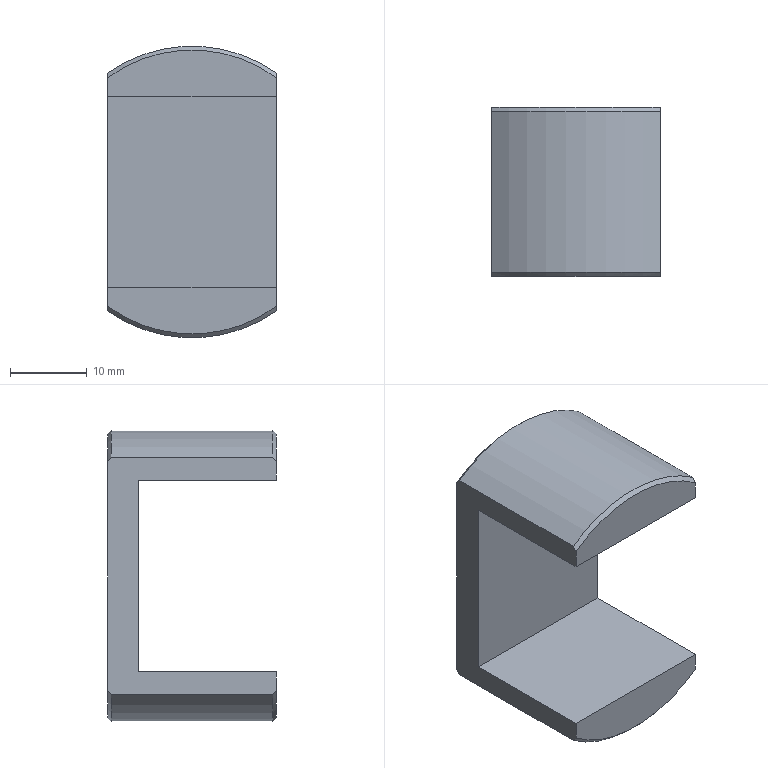Component | NX | LARGE_SLIDER | 1 solid | 14 faces | box 22 x 22 x 38 mm | volume 7394 mm3 | plane 8 | cone 4 | cylinder 2 | commonest cylinder face diameters 38 x2
STEP:
#1=CARTESIAN_POINT('',(0.,0.,0.));
#2=DIRECTION('',(0.,0.,1.));
#3=DIRECTION('',(1.,0.,0.));
#4=AXIS2_PLACEMENT_3D('',#1,#2,#3);
#5=CARTESIAN_POINT('',(-11.,-32.,-10.374));
#6=VERTEX_POINT('',#5);
#7=CARTESIAN_POINT('',(-11.,-32.,-8.));
#8=VERTEX_POINT('',#7);
#9=CARTESIAN_POINT('',(-11.,-32.,-10.992));
#10=DIRECTION('',(0.,0.,1.));
#11=VECTOR('',#10,1.);
#12=LINE('',#9,#11);
#13=CARTESIAN_POINT('',(0.,-32.,4.5));
#14=DIRECTION('',(0.,-1.,0.));
#15=DIRECTION('',(1.,0.,0.));
#16=AXIS2_PLACEMENT_3D('',#13,#14,#15);
#17=PLANE('',#16);
#18=CARTESIAN_POINT('',(-11.,-15.492));
#19=DIRECTION('',(0.,1.));
#20=VECTOR('',#19,1.);
#21=LINE('',#18,#20);
#22=(GEOMETRIC_REPRESENTATION_CONTEXT(2)PARAMETRIC_REPRESENTATION_CONTEXT()REPRESENTATION_CONTEXT('',''));
#23=DEFINITIONAL_REPRESENTATION('',(#21),#22);
#24=PCURVE('',#17,#23);
#25=CARTESIAN_POINT('',(-11.,-7.,-10.992));
#26=DIRECTION('',(1.,0.,0.));
#27=DIRECTION('',(0.,1.,0.));
#28=AXIS2_PLACEMENT_3D('',#25,#26,#27);
#29=PLANE('',#28);
#30=CARTESIAN_POINT('',(-25.,0.));
#31=DIRECTION('',(0.,1.));
#32=VECTOR('',#31,1.);
#33=LINE('',#30,#32);
#34=(GEOMETRIC_REPRESENTATION_CONTEXT(2)PARAMETRIC_REPRESENTATION_CONTEXT()REPRESENTATION_CONTEXT('',''));
#35=DEFINITIONAL_REPRESENTATION('',(#33),#34);
#36=PCURVE('',#29,#35);
#37=SURFACE_CURVE('',#12,(#24,#36),.PCURVE_S1.);
#38=EDGE_CURVE('',#6,#8,#37,.T.);
#39=ORIENTED_EDGE('',*,*,#38,.F.);
#40=CARTESIAN_POINT('',(11.,-32.,-10.374));
#41=VERTEX_POINT('',#40);
#42=CARTESIAN_POINT('',(0.,-32.,4.5));
#43=DIRECTION('',(0.,-1.,0.));
#44=DIRECTION('',(1.,0.,0.));
#45=AXIS2_PLACEMENT_3D('',#42,#43,#44);
#46=CIRCLE('',#45,18.5);
#47=CARTESIAN_POINT('',(0.,0.));
#48=DIRECTION('',(1.,0.));
#49=AXIS2_PLACEMENT_2D('',#47,#48);
#50=CIRCLE('',#49,18.5);
#51=(GEOMETRIC_REPRESENTATION_CONTEXT(2)PARAMETRIC_REPRESENTATION_CONTEXT()REPRESENTATION_CONTEXT('',''));
#52=DEFINITIONAL_REPRESENTATION('',(#50),#51);
#53=PCURVE('',#17,#52);
#54=CARTESIAN_POINT('',(0.,-31.5,4.5));
#55=DIRECTION('',(0.,1.,0.));
#56=DIRECTION('',(-1.,0.,0.));
#57=AXIS2_PLACEMENT_3D('',#54,#55,#56);
#58=CONICAL_SURFACE('',#57,19.,0.7854);
#59=CARTESIAN_POINT('',(9.425,-0.5));
#60=DIRECTION('',(-1.,0.));
#61=VECTOR('',#60,1.);
#62=LINE('',#59,#61);
#63=(GEOMETRIC_REPRESENTATION_CONTEXT(2)PARAMETRIC_REPRESENTATION_CONTEXT()REPRESENTATION_CONTEXT('',''));
#64=DEFINITIONAL_REPRESENTATION('',(#62),#63);
#65=PCURVE('',#58,#64);
#66=SURFACE_CURVE('',#46,(#53,#65),.PCURVE_S1.);
#67=EDGE_CURVE('',#6,#41,#66,.T.);
#68=ORIENTED_EDGE('',*,*,#67,.T.);
#69=CARTESIAN_POINT('',(11.,-32.,-8.));
#70=VERTEX_POINT('',#69);
#71=CARTESIAN_POINT('',(11.,-32.,19.992));
#72=DIRECTION('',(0.,0.,-1.));
#73=VECTOR('',#72,1.);
#74=LINE('',#71,#73);
#75=CARTESIAN_POINT('',(11.,15.492));
#76=DIRECTION('',(0.,-1.));
#77=VECTOR('',#76,1.);
#78=LINE('',#75,#77);
#79=(GEOMETRIC_REPRESENTATION_CONTEXT(2)PARAMETRIC_REPRESENTATION_CONTEXT()REPRESENTATION_CONTEXT('',''));
#80=DEFINITIONAL_REPRESENTATION('',(#78),#79);
#81=PCURVE('',#17,#80);
#82=CARTESIAN_POINT('',(11.,-7.,19.992));
#83=DIRECTION('',(-1.,0.,0.));
#84=DIRECTION('',(0.,-1.,0.));
#85=AXIS2_PLACEMENT_3D('',#82,#83,#84);
#86=PLANE('',#85);
#87=CARTESIAN_POINT('',(25.,0.));
#88=DIRECTION('',(0.,-1.));
#89=VECTOR('',#88,1.);
#90=LINE('',#87,#89);
#91=(GEOMETRIC_REPRESENTATION_CONTEXT(2)PARAMETRIC_REPRESENTATION_CONTEXT()REPRESENTATION_CONTEXT('',''));
#92=DEFINITIONAL_REPRESENTATION('',(#90),#91);
#93=PCURVE('',#86,#92);
#94=SURFACE_CURVE('',#74,(#81,#93),.PCURVE_S1.);
#95=EDGE_CURVE('',#70,#41,#94,.T.);
#96=ORIENTED_EDGE('',*,*,#95,.F.);
#97=CARTESIAN_POINT('',(21.,-32.,-8.));
#98=DIRECTION('',(-1.,0.,0.));
#99=VECTOR('',#98,1.);
#100=LINE('',#97,#99);
#101=CARTESIAN_POINT('',(21.,-12.5));
#102=DIRECTION('',(-1.,0.));
#103=VECTOR('',#102,1.);
#104=LINE('',#101,#103);
#105=(GEOMETRIC_REPRESENTATION_CONTEXT(2)PARAMETRIC_REPRESENTATION_CONTEXT()REPRESENTATION_CONTEXT('',''));
#106=DEFINITIONAL_REPRESENTATION('',(#104),#105);
#107=PCURVE('',#17,#106);
#108=CARTESIAN_POINT('',(21.,-14.,-8.));
#109=DIRECTION('',(0.,0.,-1.));
#110=DIRECTION('',(0.,1.,0.));
#111=AXIS2_PLACEMENT_3D('',#108,#109,#110);
#112=PLANE('',#111);
#113=CARTESIAN_POINT('',(-18.,0.));
#114=DIRECTION('',(0.,-1.));
#115=VECTOR('',#114,1.);
#116=LINE('',#113,#115);
#117=(GEOMETRIC_REPRESENTATION_CONTEXT(2)PARAMETRIC_REPRESENTATION_CONTEXT()REPRESENTATION_CONTEXT('',''));
#118=DEFINITIONAL_REPRESENTATION('',(#116),#117);
#119=PCURVE('',#112,#118);
#120=SURFACE_CURVE('',#100,(#107,#119),.PCURVE_S1.);
#121=EDGE_CURVE('',#70,#8,#120,.T.);
#122=ORIENTED_EDGE('',*,*,#121,.T.);
#123=EDGE_LOOP('',(#39,#68,#96,#122));
#124=FACE_BOUND('',#123,.T.);
#125=ADVANCED_FACE('',(#124),#17,.T.);
#126=CARTESIAN_POINT('',(-11.,-10.5,-10.992));
#127=VERTEX_POINT('',#126);
#128=CARTESIAN_POINT('',(-11.,-31.5,-10.992));
#129=VERTEX_POINT('',#128);
#130=CARTESIAN_POINT('',(-11.,-7.,-10.992));
#131=DIRECTION('',(0.,-1.,0.));
#132=VECTOR('',#131,1.);
#133=LINE('',#130,#132);
#134=CARTESIAN_POINT('',(0.,-10.,4.5));
#135=DIRECTION('',(0.,-1.,0.));
#136=DIRECTION('',(1.,0.,0.));
#137=AXIS2_PLACEMENT_3D('',#134,#135,#136);
#138=CYLINDRICAL_SURFACE('',#137,19.);
#139=CARTESIAN_POINT('',(4.095,-3.));
#140=DIRECTION('',(0.,1.));
#141=VECTOR('',#140,1.);
#142=LINE('',#139,#141);
#143=(GEOMETRIC_REPRESENTATION_CONTEXT(2)PARAMETRIC_REPRESENTATION_CONTEXT()REPRESENTATION_CONTEXT('',''));
#144=DEFINITIONAL_REPRESENTATION('',(#142),#143);
#145=PCURVE('',#138,#144);
#146=CARTESIAN_POINT('',(0.,0.));
#147=DIRECTION('',(-1.,0.));
#148=VECTOR('',#147,1.);
#149=LINE('',#146,#148);
#150=(GEOMETRIC_REPRESENTATION_CONTEXT(2)PARAMETRIC_REPRESENTATION_CONTEXT()REPRESENTATION_CONTEXT('',''));
#151=DEFINITIONAL_REPRESENTATION('',(#149),#150);
#152=PCURVE('',#29,#151);
#153=SURFACE_CURVE('',#133,(#145,#152),.PCURVE_S1.);
#154=EDGE_CURVE('',#127,#129,#153,.T.);
#155=ORIENTED_EDGE('',*,*,#154,.F.);
#156=CARTESIAN_POINT('',(11.,-10.5,-10.992));
#157=VERTEX_POINT('',#156);
#158=CARTESIAN_POINT('',(0.,-10.5,4.5));
#159=DIRECTION('',(0.,-1.,0.));
#160=DIRECTION('',(-1.,0.,0.));
#161=AXIS2_PLACEMENT_3D('',#158,#159,#160);
#162=CIRCLE('',#161,19.);
#163=CARTESIAN_POINT('',(3.142,0.5));
#164=DIRECTION('',(1.,0.));
#165=VECTOR('',#164,1.);
#166=LINE('',#163,#165);
#167=(GEOMETRIC_REPRESENTATION_CONTEXT(2)PARAMETRIC_REPRESENTATION_CONTEXT()REPRESENTATION_CONTEXT('',''));
#168=DEFINITIONAL_REPRESENTATION('',(#166),#167);
#169=PCURVE('',#138,#168);
#170=CARTESIAN_POINT('',(0.,-10.5,4.5));
#171=DIRECTION('',(0.,-1.,0.));
#172=DIRECTION('',(1.,0.,0.));
#173=AXIS2_PLACEMENT_3D('',#170,#171,#172);
#174=CONICAL_SURFACE('',#173,19.,0.7854);
#175=CARTESIAN_POINT('',(3.142,0.));
#176=DIRECTION('',(1.,-0.));
#177=VECTOR('',#176,1.);
#178=LINE('',#175,#177);
#179=(GEOMETRIC_REPRESENTATION_CONTEXT(2)PARAMETRIC_REPRESENTATION_CONTEXT()REPRESENTATION_CONTEXT('',''));
#180=DEFINITIONAL_REPRESENTATION('',(#178),#179);
#181=PCURVE('',#174,#180);
#182=SURFACE_CURVE('',#162,(#169,#181),.PCURVE_S1.);
#183=EDGE_CURVE('',#127,#157,#182,.T.);
#184=ORIENTED_EDGE('',*,*,#183,.T.);
#185=CARTESIAN_POINT('',(11.,-31.5,-10.992));
#186=VERTEX_POINT('',#185);
#187=CARTESIAN_POINT('',(11.,-7.,-10.992));
#188=DIRECTION('',(0.,-1.,0.));
#189=VECTOR('',#188,1.);
#190=LINE('',#187,#189);
#191=CARTESIAN_POINT('',(5.33,-3.));
#192=DIRECTION('',(0.,1.));
#193=VECTOR('',#192,1.);
#194=LINE('',#191,#193);
#195=(GEOMETRIC_REPRESENTATION_CONTEXT(2)PARAMETRIC_REPRESENTATION_CONTEXT()REPRESENTATION_CONTEXT('',''));
#196=DEFINITIONAL_REPRESENTATION('',(#194),#195);
#197=PCURVE('',#138,#196);
#198=CARTESIAN_POINT('',(0.,-30.984));
#199=DIRECTION('',(1.,0.));
#200=VECTOR('',#199,1.);
#201=LINE('',#198,#200);
#202=(GEOMETRIC_REPRESENTATION_CONTEXT(2)PARAMETRIC_REPRESENTATION_CONTEXT()REPRESENTATION_CONTEXT('',''));
#203=DEFINITIONAL_REPRESENTATION('',(#201),#202);
#204=PCURVE('',#86,#203);
#205=SURFACE_CURVE('',#190,(#197,#204),.PCURVE_S1.);
#206=EDGE_CURVE('',#157,#186,#205,.T.);
#207=ORIENTED_EDGE('',*,*,#206,.T.);
#208=CARTESIAN_POINT('',(0.,-31.5,4.5));
#209=DIRECTION('',(0.,1.,0.));
#210=DIRECTION('',(1.,0.,0.));
#211=AXIS2_PLACEMENT_3D('',#208,#209,#210);
#212=CIRCLE('',#211,19.);
#213=CARTESIAN_POINT('',(6.283,21.5));
#214=DIRECTION('',(-1.,0.));
#215=VECTOR('',#214,1.);
#216=LINE('',#213,#215);
#217=(GEOMETRIC_REPRESENTATION_CONTEXT(2)PARAMETRIC_REPRESENTATION_CONTEXT()REPRESENTATION_CONTEXT('',''));
#218=DEFINITIONAL_REPRESENTATION('',(#216),#217);
#219=PCURVE('',#138,#218);
#220=CARTESIAN_POINT('',(3.142,0.));
#221=DIRECTION('',(1.,-0.));
#222=VECTOR('',#221,1.);
#223=LINE('',#220,#222);
#224=(GEOMETRIC_REPRESENTATION_CONTEXT(2)PARAMETRIC_REPRESENTATION_CONTEXT()REPRESENTATION_CONTEXT('',''));
#225=DEFINITIONAL_REPRESENTATION('',(#223),#224);
#226=PCURVE('',#58,#225);
#227=SURFACE_CURVE('',#212,(#219,#226),.PCURVE_S1.);
#228=EDGE_CURVE('',#186,#129,#227,.T.);
#229=ORIENTED_EDGE('',*,*,#228,.T.);
#230=EDGE_LOOP('',(#155,#184,#207,#229));
#231=FACE_BOUND('',#230,.T.);
#232=ADVANCED_FACE('',(#231),#138,.T.);
#233=CARTESIAN_POINT('',(11.,-31.5,19.992));
#234=VERTEX_POINT('',#233);
#235=CARTESIAN_POINT('',(11.,-10.5,19.992));
#236=VERTEX_POINT('',#235);
#237=CARTESIAN_POINT('',(11.,-7.,19.992));
#238=DIRECTION('',(0.,1.,0.));
#239=VECTOR('',#238,1.);
#240=LINE('',#237,#239);
#241=CARTESIAN_POINT('',(0.,-10.,4.5));
#242=DIRECTION('',(0.,-1.,0.));
#243=DIRECTION('',(1.,0.,0.));
#244=AXIS2_PLACEMENT_3D('',#241,#242,#243);
#245=CYLINDRICAL_SURFACE('',#244,19.);
#246=CARTESIAN_POINT('',(0.9534,-3.));
#247=DIRECTION('',(0.,-1.));
#248=VECTOR('',#247,1.);
#249=LINE('',#246,#248);
#250=(GEOMETRIC_REPRESENTATION_CONTEXT(2)PARAMETRIC_REPRESENTATION_CONTEXT()REPRESENTATION_CONTEXT('',''));
#251=DEFINITIONAL_REPRESENTATION('',(#249),#250);
#252=PCURVE('',#245,#251);
#253=CARTESIAN_POINT('',(0.,0.));
#254=DIRECTION('',(-1.,0.));
#255=VECTOR('',#254,1.);
#256=LINE('',#253,#255);
#257=(GEOMETRIC_REPRESENTATION_CONTEXT(2)PARAMETRIC_REPRESENTATION_CONTEXT()REPRESENTATION_CONTEXT('',''));
#258=DEFINITIONAL_REPRESENTATION('',(#256),#257);
#259=PCURVE('',#86,#258);
#260=SURFACE_CURVE('',#240,(#252,#259),.PCURVE_S1.);
#261=EDGE_CURVE('',#234,#236,#260,.T.);
#262=ORIENTED_EDGE('',*,*,#261,.T.);
#263=CARTESIAN_POINT('',(-11.,-10.5,19.992));
#264=VERTEX_POINT('',#263);
#265=CARTESIAN_POINT('',(0.,-10.5,4.5));
#266=DIRECTION('',(0.,-1.,0.));
#267=DIRECTION('',(-1.,0.,0.));
#268=AXIS2_PLACEMENT_3D('',#265,#266,#267);
#269=CIRCLE('',#268,19.);
#270=CARTESIAN_POINT('',(-3.142,0.5));
#271=DIRECTION('',(1.,0.));
#272=VECTOR('',#271,1.);
#273=LINE('',#270,#272);
#274=(GEOMETRIC_REPRESENTATION_CONTEXT(2)PARAMETRIC_REPRESENTATION_CONTEXT()REPRESENTATION_CONTEXT('',''));
#275=DEFINITIONAL_REPRESENTATION('',(#273),#274);
#276=PCURVE('',#245,#275);
#277=CARTESIAN_POINT('',(0.,-10.5,4.5));
#278=DIRECTION('',(0.,-1.,0.));
#279=DIRECTION('',(1.,0.,0.));
#280=AXIS2_PLACEMENT_3D('',#277,#278,#279);
#281=CONICAL_SURFACE('',#280,19.,0.7854);
#282=CARTESIAN_POINT('',(-3.142,0.));
#283=DIRECTION('',(1.,0.));
#284=VECTOR('',#283,1.);
#285=LINE('',#282,#284);
#286=(GEOMETRIC_REPRESENTATION_CONTEXT(2)PARAMETRIC_REPRESENTATION_CONTEXT()REPRESENTATION_CONTEXT('',''));
#287=DEFINITIONAL_REPRESENTATION('',(#285),#286);
#288=PCURVE('',#281,#287);
#289=SURFACE_CURVE('',#269,(#276,#288),.PCURVE_S1.);
#290=EDGE_CURVE('',#236,#264,#289,.T.);
#291=ORIENTED_EDGE('',*,*,#290,.T.);
#292=CARTESIAN_POINT('',(-11.,-31.5,19.992));
#293=VERTEX_POINT('',#292);
#294=CARTESIAN_POINT('',(-11.,-7.,19.992));
#295=DIRECTION('',(0.,1.,0.));
#296=VECTOR('',#295,1.);
#297=LINE('',#294,#296);
#298=CARTESIAN_POINT('',(2.188,-3.));
#299=DIRECTION('',(0.,-1.));
#300=VECTOR('',#299,1.);
#301=LINE('',#298,#300);
#302=(GEOMETRIC_REPRESENTATION_CONTEXT(2)PARAMETRIC_REPRESENTATION_CONTEXT()REPRESENTATION_CONTEXT('',''));
#303=DEFINITIONAL_REPRESENTATION('',(#301),#302);
#304=PCURVE('',#245,#303);
#305=CARTESIAN_POINT('',(0.,30.984));
#306=DIRECTION('',(1.,0.));
#307=VECTOR('',#306,1.);
#308=LINE('',#305,#307);
#309=(GEOMETRIC_REPRESENTATION_CONTEXT(2)PARAMETRIC_REPRESENTATION_CONTEXT()REPRESENTATION_CONTEXT('',''));
#310=DEFINITIONAL_REPRESENTATION('',(#308),#309);
#311=PCURVE('',#29,#310);
#312=SURFACE_CURVE('',#297,(#304,#311),.PCURVE_S1.);
#313=EDGE_CURVE('',#293,#264,#312,.T.);
#314=ORIENTED_EDGE('',*,*,#313,.F.);
#315=CARTESIAN_POINT('',(0.,-31.5,4.5));
#316=DIRECTION('',(0.,1.,0.));
#317=DIRECTION('',(1.,0.,0.));
#318=AXIS2_PLACEMENT_3D('',#315,#316,#317);
#319=CIRCLE('',#318,19.);
#320=CARTESIAN_POINT('',(6.283,21.5));
#321=DIRECTION('',(-1.,0.));
#322=VECTOR('',#321,1.);
#323=LINE('',#320,#322);
#324=(GEOMETRIC_REPRESENTATION_CONTEXT(2)PARAMETRIC_REPRESENTATION_CONTEXT()REPRESENTATION_CONTEXT('',''));
#325=DEFINITIONAL_REPRESENTATION('',(#323),#324);
#326=PCURVE('',#245,#325);
#327=CARTESIAN_POINT('',(0.,-31.5,4.5));
#328=DIRECTION('',(0.,1.,0.));
#329=DIRECTION('',(-1.,0.,0.));
#330=AXIS2_PLACEMENT_3D('',#327,#328,#329);
#331=CONICAL_SURFACE('',#330,19.,0.7854);
#332=CARTESIAN_POINT('',(-3.142,0.));
#333=DIRECTION('',(1.,0.));
#334=VECTOR('',#333,1.);
#335=LINE('',#332,#334);
#336=(GEOMETRIC_REPRESENTATION_CONTEXT(2)PARAMETRIC_REPRESENTATION_CONTEXT()REPRESENTATION_CONTEXT('',''));
#337=DEFINITIONAL_REPRESENTATION('',(#335),#336);
#338=PCURVE('',#331,#337);
#339=SURFACE_CURVE('',#319,(#326,#338),.PCURVE_S1.);
#340=EDGE_CURVE('',#293,#234,#339,.T.);
#341=ORIENTED_EDGE('',*,*,#340,.T.);
#342=EDGE_LOOP('',(#262,#291,#314,#341));
#343=FACE_BOUND('',#342,.T.);
#344=ADVANCED_FACE('',(#343),#245,.T.);
#345=CARTESIAN_POINT('',(11.,-32.,19.374));
#346=VERTEX_POINT('',#345);
#347=CARTESIAN_POINT('',(11.,-32.,17.));
#348=VERTEX_POINT('',#347);
#349=CARTESIAN_POINT('',(11.,-32.,19.992));
#350=DIRECTION('',(0.,0.,-1.));
#351=VECTOR('',#350,1.);
#352=LINE('',#349,#351);
#353=CARTESIAN_POINT('',(0.,-32.,4.5));
#354=DIRECTION('',(0.,-1.,0.));
#355=DIRECTION('',(1.,0.,0.));
#356=AXIS2_PLACEMENT_3D('',#353,#354,#355);
#357=PLANE('',#356);
#358=CARTESIAN_POINT('',(11.,15.492));
#359=DIRECTION('',(0.,-1.));
#360=VECTOR('',#359,1.);
#361=LINE('',#358,#360);
#362=(GEOMETRIC_REPRESENTATION_CONTEXT(2)PARAMETRIC_REPRESENTATION_CONTEXT()REPRESENTATION_CONTEXT('',''));
#363=DEFINITIONAL_REPRESENTATION('',(#361),#362);
#364=PCURVE('',#357,#363);
#365=CARTESIAN_POINT('',(25.,0.));
#366=DIRECTION('',(0.,-1.));
#367=VECTOR('',#366,1.);
#368=LINE('',#365,#367);
#369=(GEOMETRIC_REPRESENTATION_CONTEXT(2)PARAMETRIC_REPRESENTATION_CONTEXT()REPRESENTATION_CONTEXT('',''));
#370=DEFINITIONAL_REPRESENTATION('',(#368),#369);
#371=PCURVE('',#86,#370);
#372=SURFACE_CURVE('',#352,(#364,#371),.PCURVE_S1.);
#373=EDGE_CURVE('',#346,#348,#372,.T.);
#374=ORIENTED_EDGE('',*,*,#373,.F.);
#375=CARTESIAN_POINT('',(-11.,-32.,19.374));
#376=VERTEX_POINT('',#375);
#377=CARTESIAN_POINT('',(0.,-32.,4.5));
#378=DIRECTION('',(0.,-1.,0.));
#379=DIRECTION('',(1.,0.,0.));
#380=AXIS2_PLACEMENT_3D('',#377,#378,#379);
#381=CIRCLE('',#380,18.5);
#382=CARTESIAN_POINT('',(0.,0.));
#383=DIRECTION('',(1.,0.));
#384=AXIS2_PLACEMENT_2D('',#382,#383);
#385=CIRCLE('',#384,18.5);
#386=(GEOMETRIC_REPRESENTATION_CONTEXT(2)PARAMETRIC_REPRESENTATION_CONTEXT()REPRESENTATION_CONTEXT('',''));
#387=DEFINITIONAL_REPRESENTATION('',(#385),#386);
#388=PCURVE('',#357,#387);
#389=CARTESIAN_POINT('',(3.142,-0.5));
#390=DIRECTION('',(-1.,0.));
#391=VECTOR('',#390,1.);
#392=LINE('',#389,#391);
#393=(GEOMETRIC_REPRESENTATION_CONTEXT(2)PARAMETRIC_REPRESENTATION_CONTEXT()REPRESENTATION_CONTEXT('',''));
#394=DEFINITIONAL_REPRESENTATION('',(#392),#393);
#395=PCURVE('',#331,#394);
#396=SURFACE_CURVE('',#381,(#388,#395),.PCURVE_S1.);
#397=EDGE_CURVE('',#346,#376,#396,.T.);
#398=ORIENTED_EDGE('',*,*,#397,.T.);
#399=CARTESIAN_POINT('',(-11.,-32.,17.));
#400=VERTEX_POINT('',#399);
#401=CARTESIAN_POINT('',(-11.,-32.,-10.992));
#402=DIRECTION('',(0.,0.,1.));
#403=VECTOR('',#402,1.);
#404=LINE('',#401,#403);
#405=CARTESIAN_POINT('',(-11.,-15.492));
#406=DIRECTION('',(0.,1.));
#407=VECTOR('',#406,1.);
#408=LINE('',#405,#407);
#409=(GEOMETRIC_REPRESENTATION_CONTEXT(2)PARAMETRIC_REPRESENTATION_CONTEXT()REPRESENTATION_CONTEXT('',''));
#410=DEFINITIONAL_REPRESENTATION('',(#408),#409);
#411=PCURVE('',#357,#410);
#412=CARTESIAN_POINT('',(-25.,0.));
#413=DIRECTION('',(0.,1.));
#414=VECTOR('',#413,1.);
#415=LINE('',#412,#414);
#416=(GEOMETRIC_REPRESENTATION_CONTEXT(2)PARAMETRIC_REPRESENTATION_CONTEXT()REPRESENTATION_CONTEXT('',''));
#417=DEFINITIONAL_REPRESENTATION('',(#415),#416);
#418=PCURVE('',#29,#417);
#419=SURFACE_CURVE('',#404,(#411,#418),.PCURVE_S1.);
#420=EDGE_CURVE('',#400,#376,#419,.T.);
#421=ORIENTED_EDGE('',*,*,#420,.F.);
#422=CARTESIAN_POINT('',(21.,-32.,17.));
#423=DIRECTION('',(-1.,0.,0.));
#424=VECTOR('',#423,1.);
#425=LINE('',#422,#424);
#426=CARTESIAN_POINT('',(21.,12.5));
#427=DIRECTION('',(-1.,0.));
#428=VECTOR('',#427,1.);
#429=LINE('',#426,#428);
#430=(GEOMETRIC_REPRESENTATION_CONTEXT(2)PARAMETRIC_REPRESENTATION_CONTEXT()REPRESENTATION_CONTEXT('',''));
#431=DEFINITIONAL_REPRESENTATION('',(#429),#430);
#432=PCURVE('',#357,#431);
#433=CARTESIAN_POINT('',(21.,-32.,17.));
#434=DIRECTION('',(0.,0.,1.));
#435=DIRECTION('',(0.,-1.,0.));
#436=AXIS2_PLACEMENT_3D('',#433,#434,#435);
#437=PLANE('',#436);
#438=CARTESIAN_POINT('',(0.,0.));
#439=DIRECTION('',(0.,-1.));
#440=VECTOR('',#439,1.);
#441=LINE('',#438,#440);
#442=(GEOMETRIC_REPRESENTATION_CONTEXT(2)PARAMETRIC_REPRESENTATION_CONTEXT()REPRESENTATION_CONTEXT('',''));
#443=DEFINITIONAL_REPRESENTATION('',(#441),#442);
#444=PCURVE('',#437,#443);
#445=SURFACE_CURVE('',#425,(#432,#444),.PCURVE_S1.);
#446=EDGE_CURVE('',#348,#400,#445,.T.);
#447=ORIENTED_EDGE('',*,*,#446,.F.);
#448=EDGE_LOOP('',(#374,#398,#421,#447));
#449=FACE_BOUND('',#448,.T.);
#450=ADVANCED_FACE('',(#449),#357,.T.);
#451=CARTESIAN_POINT('',(-11.,-10.,19.374));
#452=VERTEX_POINT('',#451);
#453=CARTESIAN_POINT('',(-11.,-10.,-10.374));
#454=VERTEX_POINT('',#453);
#455=CARTESIAN_POINT('',(-11.,-10.,4.5));
#456=DIRECTION('',(0.,0.,-1.));
#457=VECTOR('',#456,1.);
#458=LINE('',#455,#457);
#459=CARTESIAN_POINT('',(0.,-10.,4.5));
#460=DIRECTION('',(0.,1.,0.));
#461=DIRECTION('',(-1.,0.,0.));
#462=AXIS2_PLACEMENT_3D('',#459,#460,#461);
#463=PLANE('',#462);
#464=CARTESIAN_POINT('',(11.,0.));
#465=DIRECTION('',(0.,-1.));
#466=VECTOR('',#465,1.);
#467=LINE('',#464,#466);
#468=(GEOMETRIC_REPRESENTATION_CONTEXT(2)PARAMETRIC_REPRESENTATION_CONTEXT()REPRESENTATION_CONTEXT('',''));
#469=DEFINITIONAL_REPRESENTATION('',(#467),#468);
#470=PCURVE('',#463,#469);
#471=CARTESIAN_POINT('',(-3.,15.492));
#472=DIRECTION('',(0.,-1.));
#473=VECTOR('',#472,1.);
#474=LINE('',#471,#473);
#475=(GEOMETRIC_REPRESENTATION_CONTEXT(2)PARAMETRIC_REPRESENTATION_CONTEXT()REPRESENTATION_CONTEXT('',''));
#476=DEFINITIONAL_REPRESENTATION('',(#474),#475);
#477=PCURVE('',#29,#476);
#478=SURFACE_CURVE('',#458,(#470,#477),.PCURVE_S1.);
#479=EDGE_CURVE('',#452,#454,#478,.T.);
#480=ORIENTED_EDGE('',*,*,#479,.F.);
#481=CARTESIAN_POINT('',(11.,-10.,19.374));
#482=VERTEX_POINT('',#481);
#483=CARTESIAN_POINT('',(0.,-10.,4.5));
#484=DIRECTION('',(0.,1.,0.));
#485=DIRECTION('',(-1.,0.,0.));
#486=AXIS2_PLACEMENT_3D('',#483,#484,#485);
#487=CIRCLE('',#486,18.5);
#488=CARTESIAN_POINT('',(0.,0.));
#489=DIRECTION('',(1.,0.));
#490=AXIS2_PLACEMENT_2D('',#488,#489);
#491=CIRCLE('',#490,18.5);
#492=(GEOMETRIC_REPRESENTATION_CONTEXT(2)PARAMETRIC_REPRESENTATION_CONTEXT()REPRESENTATION_CONTEXT('',''));
#493=DEFINITIONAL_REPRESENTATION('',(#491),#492);
#494=PCURVE('',#463,#493);
#495=CARTESIAN_POINT('',(3.142,-0.5));
#496=DIRECTION('',(-1.,0.));
#497=VECTOR('',#496,1.);
#498=LINE('',#495,#497);
#499=(GEOMETRIC_REPRESENTATION_CONTEXT(2)PARAMETRIC_REPRESENTATION_CONTEXT()REPRESENTATION_CONTEXT('',''));
#500=DEFINITIONAL_REPRESENTATION('',(#498),#499);
#501=PCURVE('',#281,#500);
#502=SURFACE_CURVE('',#487,(#494,#501),.PCURVE_S1.);
#503=EDGE_CURVE('',#452,#482,#502,.T.);
#504=ORIENTED_EDGE('',*,*,#503,.T.);
#505=CARTESIAN_POINT('',(11.,-10.,-10.374));
#506=VERTEX_POINT('',#505);
#507=CARTESIAN_POINT('',(11.,-10.,4.5));
#508=DIRECTION('',(0.,0.,1.));
#509=VECTOR('',#508,1.);
#510=LINE('',#507,#509);
#511=CARTESIAN_POINT('',(-11.,0.));
#512=DIRECTION('',(0.,1.));
#513=VECTOR('',#512,1.);
#514=LINE('',#511,#513);
#515=(GEOMETRIC_REPRESENTATION_CONTEXT(2)PARAMETRIC_REPRESENTATION_CONTEXT()REPRESENTATION_CONTEXT('',''));
#516=DEFINITIONAL_REPRESENTATION('',(#514),#515);
#517=PCURVE('',#463,#516);
#518=CARTESIAN_POINT('',(3.,-15.492));
#519=DIRECTION('',(0.,1.));
#520=VECTOR('',#519,1.);
#521=LINE('',#518,#520);
#522=(GEOMETRIC_REPRESENTATION_CONTEXT(2)PARAMETRIC_REPRESENTATION_CONTEXT()REPRESENTATION_CONTEXT('',''));
#523=DEFINITIONAL_REPRESENTATION('',(#521),#522);
#524=PCURVE('',#86,#523);
#525=SURFACE_CURVE('',#510,(#517,#524),.PCURVE_S1.);
#526=EDGE_CURVE('',#506,#482,#525,.T.);
#527=ORIENTED_EDGE('',*,*,#526,.F.);
#528=CARTESIAN_POINT('',(0.,-10.,4.5));
#529=DIRECTION('',(0.,1.,0.));
#530=DIRECTION('',(-1.,0.,0.));
#531=AXIS2_PLACEMENT_3D('',#528,#529,#530);
#532=CIRCLE('',#531,18.5);
#533=CARTESIAN_POINT('',(0.,0.));
#534=DIRECTION('',(1.,0.));
#535=AXIS2_PLACEMENT_2D('',#533,#534);
#536=CIRCLE('',#535,18.5);
#537=(GEOMETRIC_REPRESENTATION_CONTEXT(2)PARAMETRIC_REPRESENTATION_CONTEXT()REPRESENTATION_CONTEXT('',''));
#538=DEFINITIONAL_REPRESENTATION('',(#536),#537);
#539=PCURVE('',#463,#538);
#540=CARTESIAN_POINT('',(9.425,-0.5));
#541=DIRECTION('',(-1.,0.));
#542=VECTOR('',#541,1.);
#543=LINE('',#540,#542);
#544=(GEOMETRIC_REPRESENTATION_CONTEXT(2)PARAMETRIC_REPRESENTATION_CONTEXT()REPRESENTATION_CONTEXT('',''));
#545=DEFINITIONAL_REPRESENTATION('',(#543),#544);
#546=PCURVE('',#174,#545);
#547=SURFACE_CURVE('',#532,(#539,#546),.PCURVE_S1.);
#548=EDGE_CURVE('',#506,#454,#547,.T.);
#549=ORIENTED_EDGE('',*,*,#548,.T.);
#550=EDGE_LOOP('',(#480,#504,#527,#549));
#551=FACE_BOUND('',#550,.T.);
#552=ADVANCED_FACE('',(#551),#463,.T.);
#553=ORIENTED_EDGE('',*,*,#313,.T.);
#554=CARTESIAN_POINT('',(-11.,-10.5,19.992));
#555=CARTESIAN_POINT('',(-11.,-10.333,19.787));
#556=CARTESIAN_POINT('',(-11.,-10.166,19.581));
#557=CARTESIAN_POINT('',(-11.,-10.,19.374));
#558=B_SPLINE_CURVE_WITH_KNOTS('',3,(#554,#555,#556,#557),.UNSPECIFIED.,.F.,.F.,(4,4),(0.,1.),.PIECEWISE_BEZIER_KNOTS.);
#559=CARTESIAN_POINT('',(-3.5,30.984));
#560=CARTESIAN_POINT('',(-3.333,30.779));
#561=CARTESIAN_POINT('',(-3.166,30.573));
#562=CARTESIAN_POINT('',(-3.,30.366));
#563=B_SPLINE_CURVE_WITH_KNOTS('',3,(#559,#560,#561,#562),.UNSPECIFIED.,.F.,.F.,(4,4),(0.,1.),.PIECEWISE_BEZIER_KNOTS.);
#564=(GEOMETRIC_REPRESENTATION_CONTEXT(2)PARAMETRIC_REPRESENTATION_CONTEXT()REPRESENTATION_CONTEXT('',''));
#565=DEFINITIONAL_REPRESENTATION('',(#563),#564);
#566=PCURVE('',#29,#565);
#567=CARTESIAN_POINT('',(2.188,0.));
#568=CARTESIAN_POINT('',(2.208,-0.5));
#569=B_SPLINE_CURVE_WITH_KNOTS('',1,(#567,#568),.UNSPECIFIED.,.F.,.F.,(2,2),(0.,1.),.PIECEWISE_BEZIER_KNOTS.);
#570=(GEOMETRIC_REPRESENTATION_CONTEXT(2)PARAMETRIC_REPRESENTATION_CONTEXT()REPRESENTATION_CONTEXT('',''));
#571=DEFINITIONAL_REPRESENTATION('',(#569),#570);
#572=PCURVE('',#281,#571);
#573=SURFACE_CURVE('',#558,(#566,#572),.PCURVE_S1.);
#574=EDGE_CURVE('',#264,#452,#573,.T.);
#575=ORIENTED_EDGE('',*,*,#574,.T.);
#576=ORIENTED_EDGE('',*,*,#479,.T.);
#577=CARTESIAN_POINT('',(-11.,-10.,-10.374));
#578=CARTESIAN_POINT('',(-11.,-10.166,-10.581));
#579=CARTESIAN_POINT('',(-11.,-10.333,-10.787));
#580=CARTESIAN_POINT('',(-11.,-10.5,-10.992));
#581=B_SPLINE_CURVE_WITH_KNOTS('',3,(#577,#578,#579,#580),.UNSPECIFIED.,.F.,.F.,(4,4),(0.,1.),.PIECEWISE_BEZIER_KNOTS.);
#582=CARTESIAN_POINT('',(-3.,0.6175));
#583=CARTESIAN_POINT('',(-3.166,0.4111));
#584=CARTESIAN_POINT('',(-3.333,0.2053));
#585=CARTESIAN_POINT('',(-3.5,0.));
#586=B_SPLINE_CURVE_WITH_KNOTS('',3,(#582,#583,#584,#585),.UNSPECIFIED.,.F.,.F.,(4,4),(0.,1.),.PIECEWISE_BEZIER_KNOTS.);
#587=(GEOMETRIC_REPRESENTATION_CONTEXT(2)PARAMETRIC_REPRESENTATION_CONTEXT()REPRESENTATION_CONTEXT('',''));
#588=DEFINITIONAL_REPRESENTATION('',(#586),#587);
#589=PCURVE('',#29,#588);
#590=CARTESIAN_POINT('',(4.076,-0.5));
#591=CARTESIAN_POINT('',(4.095,0.));
#592=B_SPLINE_CURVE_WITH_KNOTS('',1,(#590,#591),.UNSPECIFIED.,.F.,.F.,(2,2),(0.,1.),.PIECEWISE_BEZIER_KNOTS.);
#593=(GEOMETRIC_REPRESENTATION_CONTEXT(2)PARAMETRIC_REPRESENTATION_CONTEXT()REPRESENTATION_CONTEXT('',''));
#594=DEFINITIONAL_REPRESENTATION('',(#592),#593);
#595=PCURVE('',#174,#594);
#596=SURFACE_CURVE('',#581,(#589,#595),.PCURVE_S1.);
#597=EDGE_CURVE('',#454,#127,#596,.T.);
#598=ORIENTED_EDGE('',*,*,#597,.T.);
#599=ORIENTED_EDGE('',*,*,#154,.T.);
#600=CARTESIAN_POINT('',(-11.,-31.5,-10.992));
#601=CARTESIAN_POINT('',(-11.,-31.667,-10.787));
#602=CARTESIAN_POINT('',(-11.,-31.834,-10.581));
#603=CARTESIAN_POINT('',(-11.,-32.,-10.374));
#604=B_SPLINE_CURVE_WITH_KNOTS('',3,(#600,#601,#602,#603),.UNSPECIFIED.,.F.,.F.,(4,4),(0.,1.),.PIECEWISE_BEZIER_KNOTS.);
#605=CARTESIAN_POINT('',(-24.5,0.));
#606=CARTESIAN_POINT('',(-24.667,0.2053));
#607=CARTESIAN_POINT('',(-24.834,0.4111));
#608=CARTESIAN_POINT('',(-25.,0.6175));
#609=B_SPLINE_CURVE_WITH_KNOTS('',3,(#605,#606,#607,#608),.UNSPECIFIED.,.F.,.F.,(4,4),(0.,1.),.PIECEWISE_BEZIER_KNOTS.);
#610=(GEOMETRIC_REPRESENTATION_CONTEXT(2)PARAMETRIC_REPRESENTATION_CONTEXT()REPRESENTATION_CONTEXT('',''));
#611=DEFINITIONAL_REPRESENTATION('',(#609),#610);
#612=PCURVE('',#29,#611);
#613=CARTESIAN_POINT('',(5.33,0.));
#614=CARTESIAN_POINT('',(5.349,-0.5));
#615=B_SPLINE_CURVE_WITH_KNOTS('',1,(#613,#614),.UNSPECIFIED.,.F.,.F.,(2,2),(0.,1.),.PIECEWISE_BEZIER_KNOTS.);
#616=(GEOMETRIC_REPRESENTATION_CONTEXT(2)PARAMETRIC_REPRESENTATION_CONTEXT()REPRESENTATION_CONTEXT('',''));
#617=DEFINITIONAL_REPRESENTATION('',(#615),#616);
#618=PCURVE('',#58,#617);
#619=SURFACE_CURVE('',#604,(#612,#618),.PCURVE_S1.);
#620=EDGE_CURVE('',#129,#6,#619,.T.);
#621=ORIENTED_EDGE('',*,*,#620,.T.);
#622=ORIENTED_EDGE('',*,*,#38,.T.);
#623=CARTESIAN_POINT('',(-11.,-14.,-8.));
#624=VERTEX_POINT('',#623);
#625=CARTESIAN_POINT('',(-11.,-7.,-8.));
#626=DIRECTION('',(0.,1.,0.));
#627=VECTOR('',#626,1.);
#628=LINE('',#625,#627);
#629=CARTESIAN_POINT('',(0.,2.992));
#630=DIRECTION('',(1.,0.));
#631=VECTOR('',#630,1.);
#632=LINE('',#629,#631);
#633=(GEOMETRIC_REPRESENTATION_CONTEXT(2)PARAMETRIC_REPRESENTATION_CONTEXT()REPRESENTATION_CONTEXT('',''));
#634=DEFINITIONAL_REPRESENTATION('',(#632),#633);
#635=PCURVE('',#29,#634);
#636=CARTESIAN_POINT('',(7.,-32.));
#637=DIRECTION('',(1.,0.));
#638=VECTOR('',#637,1.);
#639=LINE('',#636,#638);
#640=(GEOMETRIC_REPRESENTATION_CONTEXT(2)PARAMETRIC_REPRESENTATION_CONTEXT()REPRESENTATION_CONTEXT('',''));
#641=DEFINITIONAL_REPRESENTATION('',(#639),#640);
#642=PCURVE('',#112,#641);
#643=SURFACE_CURVE('',#628,(#635,#642),.PCURVE_S1.);
#644=EDGE_CURVE('',#8,#624,#643,.T.);
#645=ORIENTED_EDGE('',*,*,#644,.T.);
#646=CARTESIAN_POINT('',(-11.,-14.,17.));
#647=VERTEX_POINT('',#646);
#648=CARTESIAN_POINT('',(-11.,-14.,-10.992));
#649=DIRECTION('',(0.,0.,1.));
#650=VECTOR('',#649,1.);
#651=LINE('',#648,#650);
#652=CARTESIAN_POINT('',(-7.,0.));
#653=DIRECTION('',(0.,1.));
#654=VECTOR('',#653,1.);
#655=LINE('',#652,#654);
#656=(GEOMETRIC_REPRESENTATION_CONTEXT(2)PARAMETRIC_REPRESENTATION_CONTEXT()REPRESENTATION_CONTEXT('',''));
#657=DEFINITIONAL_REPRESENTATION('',(#655),#656);
#658=PCURVE('',#29,#657);
#659=CARTESIAN_POINT('',(21.,-14.,17.));
#660=DIRECTION('',(0.,1.,0.));
#661=DIRECTION('',(-1.,0.,0.));
#662=AXIS2_PLACEMENT_3D('',#659,#660,#661);
#663=PLANE('',#662);
#664=CARTESIAN_POINT('',(32.,-27.992));
#665=DIRECTION('',(0.,1.));
#666=VECTOR('',#665,1.);
#667=LINE('',#664,#666);
#668=(GEOMETRIC_REPRESENTATION_CONTEXT(2)PARAMETRIC_REPRESENTATION_CONTEXT()REPRESENTATION_CONTEXT('',''));
#669=DEFINITIONAL_REPRESENTATION('',(#667),#668);
#670=PCURVE('',#663,#669);
#671=SURFACE_CURVE('',#651,(#658,#670),.PCURVE_S1.);
#672=EDGE_CURVE('',#624,#647,#671,.T.);
#673=ORIENTED_EDGE('',*,*,#672,.T.);
#674=CARTESIAN_POINT('',(-11.,-7.,17.));
#675=DIRECTION('',(0.,-1.,0.));
#676=VECTOR('',#675,1.);
#677=LINE('',#674,#676);
#678=CARTESIAN_POINT('',(0.,27.992));
#679=DIRECTION('',(-1.,0.));
#680=VECTOR('',#679,1.);
#681=LINE('',#678,#680);
#682=(GEOMETRIC_REPRESENTATION_CONTEXT(2)PARAMETRIC_REPRESENTATION_CONTEXT()REPRESENTATION_CONTEXT('',''));
#683=DEFINITIONAL_REPRESENTATION('',(#681),#682);
#684=PCURVE('',#29,#683);
#685=CARTESIAN_POINT('',(-25.,-32.));
#686=DIRECTION('',(1.,0.));
#687=VECTOR('',#686,1.);
#688=LINE('',#685,#687);
#689=(GEOMETRIC_REPRESENTATION_CONTEXT(2)PARAMETRIC_REPRESENTATION_CONTEXT()REPRESENTATION_CONTEXT('',''));
#690=DEFINITIONAL_REPRESENTATION('',(#688),#689);
#691=PCURVE('',#437,#690);
#692=SURFACE_CURVE('',#677,(#684,#691),.PCURVE_S1.);
#693=EDGE_CURVE('',#647,#400,#692,.T.);
#694=ORIENTED_EDGE('',*,*,#693,.T.);
#695=ORIENTED_EDGE('',*,*,#420,.T.);
#696=CARTESIAN_POINT('',(-11.,-32.,19.374));
#697=CARTESIAN_POINT('',(-11.,-31.834,19.581));
#698=CARTESIAN_POINT('',(-11.,-31.667,19.787));
#699=CARTESIAN_POINT('',(-11.,-31.5,19.992));
#700=B_SPLINE_CURVE_WITH_KNOTS('',3,(#696,#697,#698,#699),.UNSPECIFIED.,.F.,.F.,(4,4),(0.,1.),.PIECEWISE_BEZIER_KNOTS.);
#701=CARTESIAN_POINT('',(-25.,30.366));
#702=CARTESIAN_POINT('',(-24.834,30.573));
#703=CARTESIAN_POINT('',(-24.667,30.779));
#704=CARTESIAN_POINT('',(-24.5,30.984));
#705=B_SPLINE_CURVE_WITH_KNOTS('',3,(#701,#702,#703,#704),.UNSPECIFIED.,.F.,.F.,(4,4),(0.,1.),.PIECEWISE_BEZIER_KNOTS.);
#706=(GEOMETRIC_REPRESENTATION_CONTEXT(2)PARAMETRIC_REPRESENTATION_CONTEXT()REPRESENTATION_CONTEXT('',''));
#707=DEFINITIONAL_REPRESENTATION('',(#705),#706);
#708=PCURVE('',#29,#707);
#709=CARTESIAN_POINT('',(0.934,-0.5));
#710=CARTESIAN_POINT('',(0.9534,0.));
#711=B_SPLINE_CURVE_WITH_KNOTS('',1,(#709,#710),.UNSPECIFIED.,.F.,.F.,(2,2),(0.,1.),.PIECEWISE_BEZIER_KNOTS.);
#712=(GEOMETRIC_REPRESENTATION_CONTEXT(2)PARAMETRIC_REPRESENTATION_CONTEXT()REPRESENTATION_CONTEXT('',''));
#713=DEFINITIONAL_REPRESENTATION('',(#711),#712);
#714=PCURVE('',#331,#713);
#715=SURFACE_CURVE('',#700,(#708,#714),.PCURVE_S1.);
#716=EDGE_CURVE('',#376,#293,#715,.T.);
#717=ORIENTED_EDGE('',*,*,#716,.T.);
#718=EDGE_LOOP('',(#553,#575,#576,#598,#599,#621,#622,#645,#673,#694,#695,#717));
#719=FACE_BOUND('',#718,.T.);
#720=ADVANCED_FACE('',(#719),#29,.F.);
#721=ORIENTED_EDGE('',*,*,#526,.T.);
#722=CARTESIAN_POINT('',(11.,-10.,19.374));
#723=CARTESIAN_POINT('',(11.,-10.166,19.581));
#724=CARTESIAN_POINT('',(11.,-10.333,19.787));
#725=CARTESIAN_POINT('',(11.,-10.5,19.992));
#726=B_SPLINE_CURVE_WITH_KNOTS('',3,(#722,#723,#724,#725),.UNSPECIFIED.,.F.,.F.,(4,4),(0.,1.),.PIECEWISE_BEZIER_KNOTS.);
#727=CARTESIAN_POINT('',(3.,-0.6175));
#728=CARTESIAN_POINT('',(3.166,-0.4111));
#729=CARTESIAN_POINT('',(3.333,-0.2053));
#730=CARTESIAN_POINT('',(3.5,0.));
#731=B_SPLINE_CURVE_WITH_KNOTS('',3,(#727,#728,#729,#730),.UNSPECIFIED.,.F.,.F.,(4,4),(0.,1.),.PIECEWISE_BEZIER_KNOTS.);
#732=(GEOMETRIC_REPRESENTATION_CONTEXT(2)PARAMETRIC_REPRESENTATION_CONTEXT()REPRESENTATION_CONTEXT('',''));
#733=DEFINITIONAL_REPRESENTATION('',(#731),#732);
#734=PCURVE('',#86,#733);
#735=CARTESIAN_POINT('',(0.934,-0.5));
#736=CARTESIAN_POINT('',(0.9534,0.));
#737=B_SPLINE_CURVE_WITH_KNOTS('',1,(#735,#736),.UNSPECIFIED.,.F.,.F.,(2,2),(0.,1.),.PIECEWISE_BEZIER_KNOTS.);
#738=(GEOMETRIC_REPRESENTATION_CONTEXT(2)PARAMETRIC_REPRESENTATION_CONTEXT()REPRESENTATION_CONTEXT('',''));
#739=DEFINITIONAL_REPRESENTATION('',(#737),#738);
#740=PCURVE('',#281,#739);
#741=SURFACE_CURVE('',#726,(#734,#740),.PCURVE_S1.);
#742=EDGE_CURVE('',#482,#236,#741,.T.);
#743=ORIENTED_EDGE('',*,*,#742,.T.);
#744=ORIENTED_EDGE('',*,*,#261,.F.);
#745=CARTESIAN_POINT('',(11.,-31.5,19.992));
#746=CARTESIAN_POINT('',(11.,-31.667,19.787));
#747=CARTESIAN_POINT('',(11.,-31.834,19.581));
#748=CARTESIAN_POINT('',(11.,-32.,19.374));
#749=B_SPLINE_CURVE_WITH_KNOTS('',3,(#745,#746,#747,#748),.UNSPECIFIED.,.F.,.F.,(4,4),(0.,1.),.PIECEWISE_BEZIER_KNOTS.);
#750=CARTESIAN_POINT('',(24.5,0.));
#751=CARTESIAN_POINT('',(24.667,-0.2053));
#752=CARTESIAN_POINT('',(24.834,-0.4111));
#753=CARTESIAN_POINT('',(25.,-0.6175));
#754=B_SPLINE_CURVE_WITH_KNOTS('',3,(#750,#751,#752,#753),.UNSPECIFIED.,.F.,.F.,(4,4),(0.,1.),.PIECEWISE_BEZIER_KNOTS.);
#755=(GEOMETRIC_REPRESENTATION_CONTEXT(2)PARAMETRIC_REPRESENTATION_CONTEXT()REPRESENTATION_CONTEXT('',''));
#756=DEFINITIONAL_REPRESENTATION('',(#754),#755);
#757=PCURVE('',#86,#756);
#758=CARTESIAN_POINT('',(2.188,0.));
#759=CARTESIAN_POINT('',(2.208,-0.5));
#760=B_SPLINE_CURVE_WITH_KNOTS('',1,(#758,#759),.UNSPECIFIED.,.F.,.F.,(2,2),(0.,1.),.PIECEWISE_BEZIER_KNOTS.);
#761=(GEOMETRIC_REPRESENTATION_CONTEXT(2)PARAMETRIC_REPRESENTATION_CONTEXT()REPRESENTATION_CONTEXT('',''));
#762=DEFINITIONAL_REPRESENTATION('',(#760),#761);
#763=PCURVE('',#331,#762);
#764=SURFACE_CURVE('',#749,(#757,#763),.PCURVE_S1.);
#765=EDGE_CURVE('',#234,#346,#764,.T.);
#766=ORIENTED_EDGE('',*,*,#765,.T.);
#767=ORIENTED_EDGE('',*,*,#373,.T.);
#768=CARTESIAN_POINT('',(11.,-14.,17.));
#769=VERTEX_POINT('',#768);
#770=CARTESIAN_POINT('',(11.,-7.,17.));
#771=DIRECTION('',(0.,1.,0.));
#772=VECTOR('',#771,1.);
#773=LINE('',#770,#772);
#774=CARTESIAN_POINT('',(0.,-2.992));
#775=DIRECTION('',(-1.,0.));
#776=VECTOR('',#775,1.);
#777=LINE('',#774,#776);
#778=(GEOMETRIC_REPRESENTATION_CONTEXT(2)PARAMETRIC_REPRESENTATION_CONTEXT()REPRESENTATION_CONTEXT('',''));
#779=DEFINITIONAL_REPRESENTATION('',(#777),#778);
#780=PCURVE('',#86,#779);
#781=CARTESIAN_POINT('',(-25.,-10.));
#782=DIRECTION('',(-1.,0.));
#783=VECTOR('',#782,1.);
#784=LINE('',#781,#783);
#785=(GEOMETRIC_REPRESENTATION_CONTEXT(2)PARAMETRIC_REPRESENTATION_CONTEXT()REPRESENTATION_CONTEXT('',''));
#786=DEFINITIONAL_REPRESENTATION('',(#784),#785);
#787=PCURVE('',#437,#786);
#788=SURFACE_CURVE('',#773,(#780,#787),.PCURVE_S1.);
#789=EDGE_CURVE('',#348,#769,#788,.T.);
#790=ORIENTED_EDGE('',*,*,#789,.T.);
#791=CARTESIAN_POINT('',(11.,-14.,-8.));
#792=VERTEX_POINT('',#791);
#793=CARTESIAN_POINT('',(11.,-14.,19.992));
#794=DIRECTION('',(0.,0.,-1.));
#795=VECTOR('',#794,1.);
#796=LINE('',#793,#795);
#797=CARTESIAN_POINT('',(7.,0.));
#798=DIRECTION('',(0.,-1.));
#799=VECTOR('',#798,1.);
#800=LINE('',#797,#799);
#801=(GEOMETRIC_REPRESENTATION_CONTEXT(2)PARAMETRIC_REPRESENTATION_CONTEXT()REPRESENTATION_CONTEXT('',''));
#802=DEFINITIONAL_REPRESENTATION('',(#800),#801);
#803=PCURVE('',#86,#802);
#804=CARTESIAN_POINT('',(10.,2.992));
#805=DIRECTION('',(0.,-1.));
#806=VECTOR('',#805,1.);
#807=LINE('',#804,#806);
#808=(GEOMETRIC_REPRESENTATION_CONTEXT(2)PARAMETRIC_REPRESENTATION_CONTEXT()REPRESENTATION_CONTEXT('',''));
#809=DEFINITIONAL_REPRESENTATION('',(#807),#808);
#810=PCURVE('',#663,#809);
#811=SURFACE_CURVE('',#796,(#803,#810),.PCURVE_S1.);
#812=EDGE_CURVE('',#769,#792,#811,.T.);
#813=ORIENTED_EDGE('',*,*,#812,.T.);
#814=CARTESIAN_POINT('',(11.,-7.,-8.));
#815=DIRECTION('',(0.,-1.,0.));
#816=VECTOR('',#815,1.);
#817=LINE('',#814,#816);
#818=CARTESIAN_POINT('',(0.,-27.992));
#819=DIRECTION('',(1.,0.));
#820=VECTOR('',#819,1.);
#821=LINE('',#818,#820);
#822=(GEOMETRIC_REPRESENTATION_CONTEXT(2)PARAMETRIC_REPRESENTATION_CONTEXT()REPRESENTATION_CONTEXT('',''));
#823=DEFINITIONAL_REPRESENTATION('',(#821),#822);
#824=PCURVE('',#86,#823);
#825=CARTESIAN_POINT('',(7.,-10.));
#826=DIRECTION('',(-1.,0.));
#827=VECTOR('',#826,1.);
#828=LINE('',#825,#827);
#829=(GEOMETRIC_REPRESENTATION_CONTEXT(2)PARAMETRIC_REPRESENTATION_CONTEXT()REPRESENTATION_CONTEXT('',''));
#830=DEFINITIONAL_REPRESENTATION('',(#828),#829);
#831=PCURVE('',#112,#830);
#832=SURFACE_CURVE('',#817,(#824,#831),.PCURVE_S1.);
#833=EDGE_CURVE('',#792,#70,#832,.T.);
#834=ORIENTED_EDGE('',*,*,#833,.T.);
#835=ORIENTED_EDGE('',*,*,#95,.T.);
#836=CARTESIAN_POINT('',(11.,-32.,-10.374));
#837=CARTESIAN_POINT('',(11.,-31.834,-10.581));
#838=CARTESIAN_POINT('',(11.,-31.667,-10.787));
#839=CARTESIAN_POINT('',(11.,-31.5,-10.992));
#840=B_SPLINE_CURVE_WITH_KNOTS('',3,(#836,#837,#838,#839),.UNSPECIFIED.,.F.,.F.,(4,4),(0.,1.),.PIECEWISE_BEZIER_KNOTS.);
#841=CARTESIAN_POINT('',(25.,-30.366));
#842=CARTESIAN_POINT('',(24.834,-30.573));
#843=CARTESIAN_POINT('',(24.667,-30.779));
#844=CARTESIAN_POINT('',(24.5,-30.984));
#845=B_SPLINE_CURVE_WITH_KNOTS('',3,(#841,#842,#843,#844),.UNSPECIFIED.,.F.,.F.,(4,4),(0.,1.),.PIECEWISE_BEZIER_KNOTS.);
#846=(GEOMETRIC_REPRESENTATION_CONTEXT(2)PARAMETRIC_REPRESENTATION_CONTEXT()REPRESENTATION_CONTEXT('',''));
#847=DEFINITIONAL_REPRESENTATION('',(#845),#846);
#848=PCURVE('',#86,#847);
#849=CARTESIAN_POINT('',(4.076,-0.5));
#850=CARTESIAN_POINT('',(4.095,0.));
#851=B_SPLINE_CURVE_WITH_KNOTS('',1,(#849,#850),.UNSPECIFIED.,.F.,.F.,(2,2),(0.,1.),.PIECEWISE_BEZIER_KNOTS.);
#852=(GEOMETRIC_REPRESENTATION_CONTEXT(2)PARAMETRIC_REPRESENTATION_CONTEXT()REPRESENTATION_CONTEXT('',''));
#853=DEFINITIONAL_REPRESENTATION('',(#851),#852);
#854=PCURVE('',#58,#853);
#855=SURFACE_CURVE('',#840,(#848,#854),.PCURVE_S1.);
#856=EDGE_CURVE('',#41,#186,#855,.T.);
#857=ORIENTED_EDGE('',*,*,#856,.T.);
#858=ORIENTED_EDGE('',*,*,#206,.F.);
#859=CARTESIAN_POINT('',(11.,-10.5,-10.992));
#860=CARTESIAN_POINT('',(11.,-10.333,-10.787));
#861=CARTESIAN_POINT('',(11.,-10.166,-10.581));
#862=CARTESIAN_POINT('',(11.,-10.,-10.374));
#863=B_SPLINE_CURVE_WITH_KNOTS('',3,(#859,#860,#861,#862),.UNSPECIFIED.,.F.,.F.,(4,4),(0.,1.),.PIECEWISE_BEZIER_KNOTS.);
#864=CARTESIAN_POINT('',(3.5,-30.984));
#865=CARTESIAN_POINT('',(3.333,-30.779));
#866=CARTESIAN_POINT('',(3.166,-30.573));
#867=CARTESIAN_POINT('',(3.,-30.366));
#868=B_SPLINE_CURVE_WITH_KNOTS('',3,(#864,#865,#866,#867),.UNSPECIFIED.,.F.,.F.,(4,4),(0.,1.),.PIECEWISE_BEZIER_KNOTS.);
#869=(GEOMETRIC_REPRESENTATION_CONTEXT(2)PARAMETRIC_REPRESENTATION_CONTEXT()REPRESENTATION_CONTEXT('',''));
#870=DEFINITIONAL_REPRESENTATION('',(#868),#869);
#871=PCURVE('',#86,#870);
#872=CARTESIAN_POINT('',(5.33,0.));
#873=CARTESIAN_POINT('',(5.349,-0.5));
#874=B_SPLINE_CURVE_WITH_KNOTS('',1,(#872,#873),.UNSPECIFIED.,.F.,.F.,(2,2),(0.,1.),.PIECEWISE_BEZIER_KNOTS.);
#875=(GEOMETRIC_REPRESENTATION_CONTEXT(2)PARAMETRIC_REPRESENTATION_CONTEXT()REPRESENTATION_CONTEXT('',''));
#876=DEFINITIONAL_REPRESENTATION('',(#874),#875);
#877=PCURVE('',#174,#876);
#878=SURFACE_CURVE('',#863,(#871,#877),.PCURVE_S1.);
#879=EDGE_CURVE('',#157,#506,#878,.T.);
#880=ORIENTED_EDGE('',*,*,#879,.T.);
#881=EDGE_LOOP('',(#721,#743,#744,#766,#767,#790,#813,#834,#835,#857,#858,#880));
#882=FACE_BOUND('',#881,.T.);
#883=ADVANCED_FACE('',(#882),#86,.F.);
#884=ORIENTED_EDGE('',*,*,#121,.F.);
#885=ORIENTED_EDGE('',*,*,#833,.F.);
#886=CARTESIAN_POINT('',(21.,-14.,-8.));
#887=DIRECTION('',(1.,0.,0.));
#888=VECTOR('',#887,1.);
#889=LINE('',#886,#888);
#890=CARTESIAN_POINT('',(0.,0.));
#891=DIRECTION('',(0.,1.));
#892=VECTOR('',#891,1.);
#893=LINE('',#890,#892);
#894=(GEOMETRIC_REPRESENTATION_CONTEXT(2)PARAMETRIC_REPRESENTATION_CONTEXT()REPRESENTATION_CONTEXT('',''));
#895=DEFINITIONAL_REPRESENTATION('',(#893),#894);
#896=PCURVE('',#112,#895);
#897=CARTESIAN_POINT('',(0.,-25.));
#898=DIRECTION('',(-1.,0.));
#899=VECTOR('',#898,1.);
#900=LINE('',#897,#899);
#901=(GEOMETRIC_REPRESENTATION_CONTEXT(2)PARAMETRIC_REPRESENTATION_CONTEXT()REPRESENTATION_CONTEXT('',''));
#902=DEFINITIONAL_REPRESENTATION('',(#900),#901);
#903=PCURVE('',#663,#902);
#904=SURFACE_CURVE('',#889,(#896,#903),.PCURVE_S1.);
#905=EDGE_CURVE('',#624,#792,#904,.T.);
#906=ORIENTED_EDGE('',*,*,#905,.F.);
#907=ORIENTED_EDGE('',*,*,#644,.F.);
#908=EDGE_LOOP('',(#884,#885,#906,#907));
#909=FACE_BOUND('',#908,.T.);
#910=ADVANCED_FACE('',(#909),#112,.F.);
#911=CARTESIAN_POINT('',(21.,-14.,17.));
#912=DIRECTION('',(1.,0.,0.));
#913=VECTOR('',#912,1.);
#914=LINE('',#911,#913);
#915=CARTESIAN_POINT('',(-18.,0.));
#916=DIRECTION('',(0.,1.));
#917=VECTOR('',#916,1.);
#918=LINE('',#915,#917);
#919=(GEOMETRIC_REPRESENTATION_CONTEXT(2)PARAMETRIC_REPRESENTATION_CONTEXT()REPRESENTATION_CONTEXT('',''));
#920=DEFINITIONAL_REPRESENTATION('',(#918),#919);
#921=PCURVE('',#437,#920);
#922=CARTESIAN_POINT('',(0.,0.));
#923=DIRECTION('',(-1.,0.));
#924=VECTOR('',#923,1.);
#925=LINE('',#922,#924);
#926=(GEOMETRIC_REPRESENTATION_CONTEXT(2)PARAMETRIC_REPRESENTATION_CONTEXT()REPRESENTATION_CONTEXT('',''));
#927=DEFINITIONAL_REPRESENTATION('',(#925),#926);
#928=PCURVE('',#663,#927);
#929=SURFACE_CURVE('',#914,(#921,#928),.PCURVE_S1.);
#930=EDGE_CURVE('',#647,#769,#929,.T.);
#931=ORIENTED_EDGE('',*,*,#930,.T.);
#932=ORIENTED_EDGE('',*,*,#789,.F.);
#933=ORIENTED_EDGE('',*,*,#446,.T.);
#934=ORIENTED_EDGE('',*,*,#693,.F.);
#935=EDGE_LOOP('',(#931,#932,#933,#934));
#936=FACE_BOUND('',#935,.T.);
#937=ADVANCED_FACE('',(#936),#437,.F.);
#938=ORIENTED_EDGE('',*,*,#905,.T.);
#939=ORIENTED_EDGE('',*,*,#812,.F.);
#940=ORIENTED_EDGE('',*,*,#930,.F.);
#941=ORIENTED_EDGE('',*,*,#672,.F.);
#942=EDGE_LOOP('',(#938,#939,#940,#941));
#943=FACE_BOUND('',#942,.T.);
#944=ADVANCED_FACE('',(#943),#663,.F.);
#945=ORIENTED_EDGE('',*,*,#742,.F.);
#946=ORIENTED_EDGE('',*,*,#503,.F.);
#947=ORIENTED_EDGE('',*,*,#574,.F.);
#948=ORIENTED_EDGE('',*,*,#290,.F.);
#949=EDGE_LOOP('',(#945,#946,#947,#948));
#950=FACE_BOUND('',#949,.T.);
#951=ADVANCED_FACE('',(#950),#281,.T.);
#952=ORIENTED_EDGE('',*,*,#597,.F.);
#953=ORIENTED_EDGE('',*,*,#548,.F.);
#954=ORIENTED_EDGE('',*,*,#879,.F.);
#955=ORIENTED_EDGE('',*,*,#183,.F.);
#956=EDGE_LOOP('',(#952,#953,#954,#955));
#957=FACE_BOUND('',#956,.T.);
#958=ADVANCED_FACE('',(#957),#174,.T.);
#959=ORIENTED_EDGE('',*,*,#716,.F.);
#960=ORIENTED_EDGE('',*,*,#397,.F.);
#961=ORIENTED_EDGE('',*,*,#765,.F.);
#962=ORIENTED_EDGE('',*,*,#340,.F.);
#963=EDGE_LOOP('',(#959,#960,#961,#962));
#964=FACE_BOUND('',#963,.T.);
#965=ADVANCED_FACE('',(#964),#331,.T.);
#966=ORIENTED_EDGE('',*,*,#856,.F.);
#967=ORIENTED_EDGE('',*,*,#67,.F.);
#968=ORIENTED_EDGE('',*,*,#620,.F.);
#969=ORIENTED_EDGE('',*,*,#228,.F.);
#970=EDGE_LOOP('',(#966,#967,#968,#969));
#971=FACE_BOUND('',#970,.T.);
#972=ADVANCED_FACE('',(#971),#58,.T.);
#973=CLOSED_SHELL('',(#125,#232,#344,#450,#552,#720,#883,#910,#937,#944,#951,#958,#965,#972));
#974=MANIFOLD_SOLID_BREP('',#973);
#975=(LENGTH_UNIT()NAMED_UNIT(*)SI_UNIT(.MILLI.,.METRE.));
#976=UNCERTAINTY_MEASURE_WITH_UNIT(LENGTH_MEASURE(0.002),#975,'','');
#977=(NAMED_UNIT(*)PLANE_ANGLE_UNIT()SI_UNIT($,.RADIAN.));
#978=(NAMED_UNIT(*)SI_UNIT($,.STERADIAN.)SOLID_ANGLE_UNIT());
#979=(GEOMETRIC_REPRESENTATION_CONTEXT(3)GLOBAL_UNCERTAINTY_ASSIGNED_CONTEXT((#976))GLOBAL_UNIT_ASSIGNED_CONTEXT((#975,#977,#978))REPRESENTATION_CONTEXT('',''));
#980=ADVANCED_BREP_SHAPE_REPRESENTATION('',(#4,#974),#979);